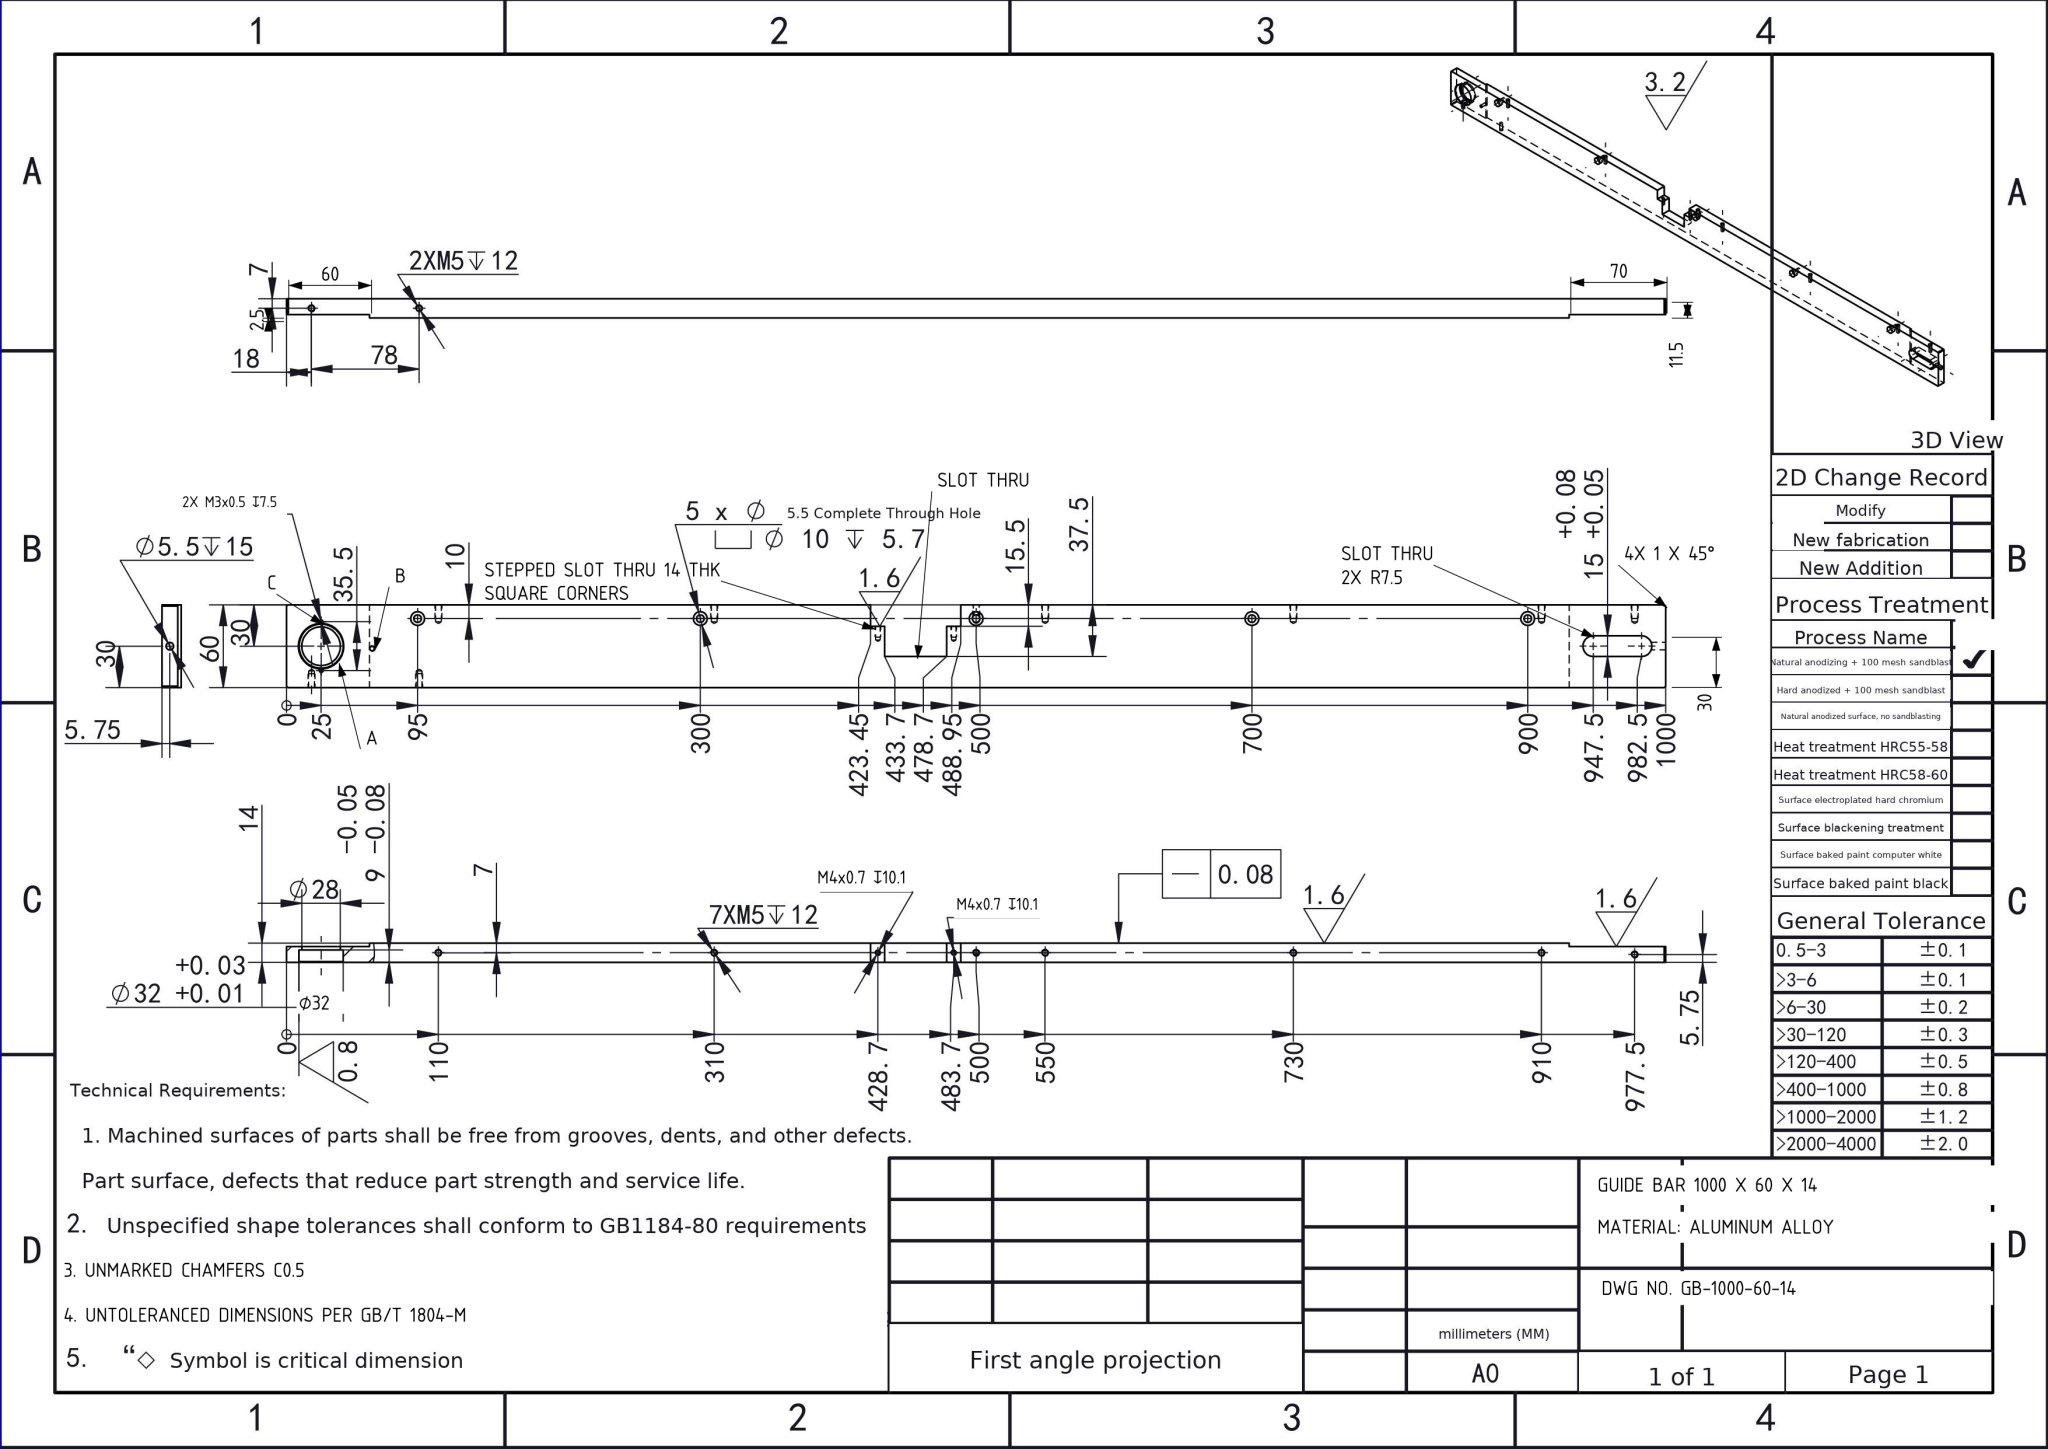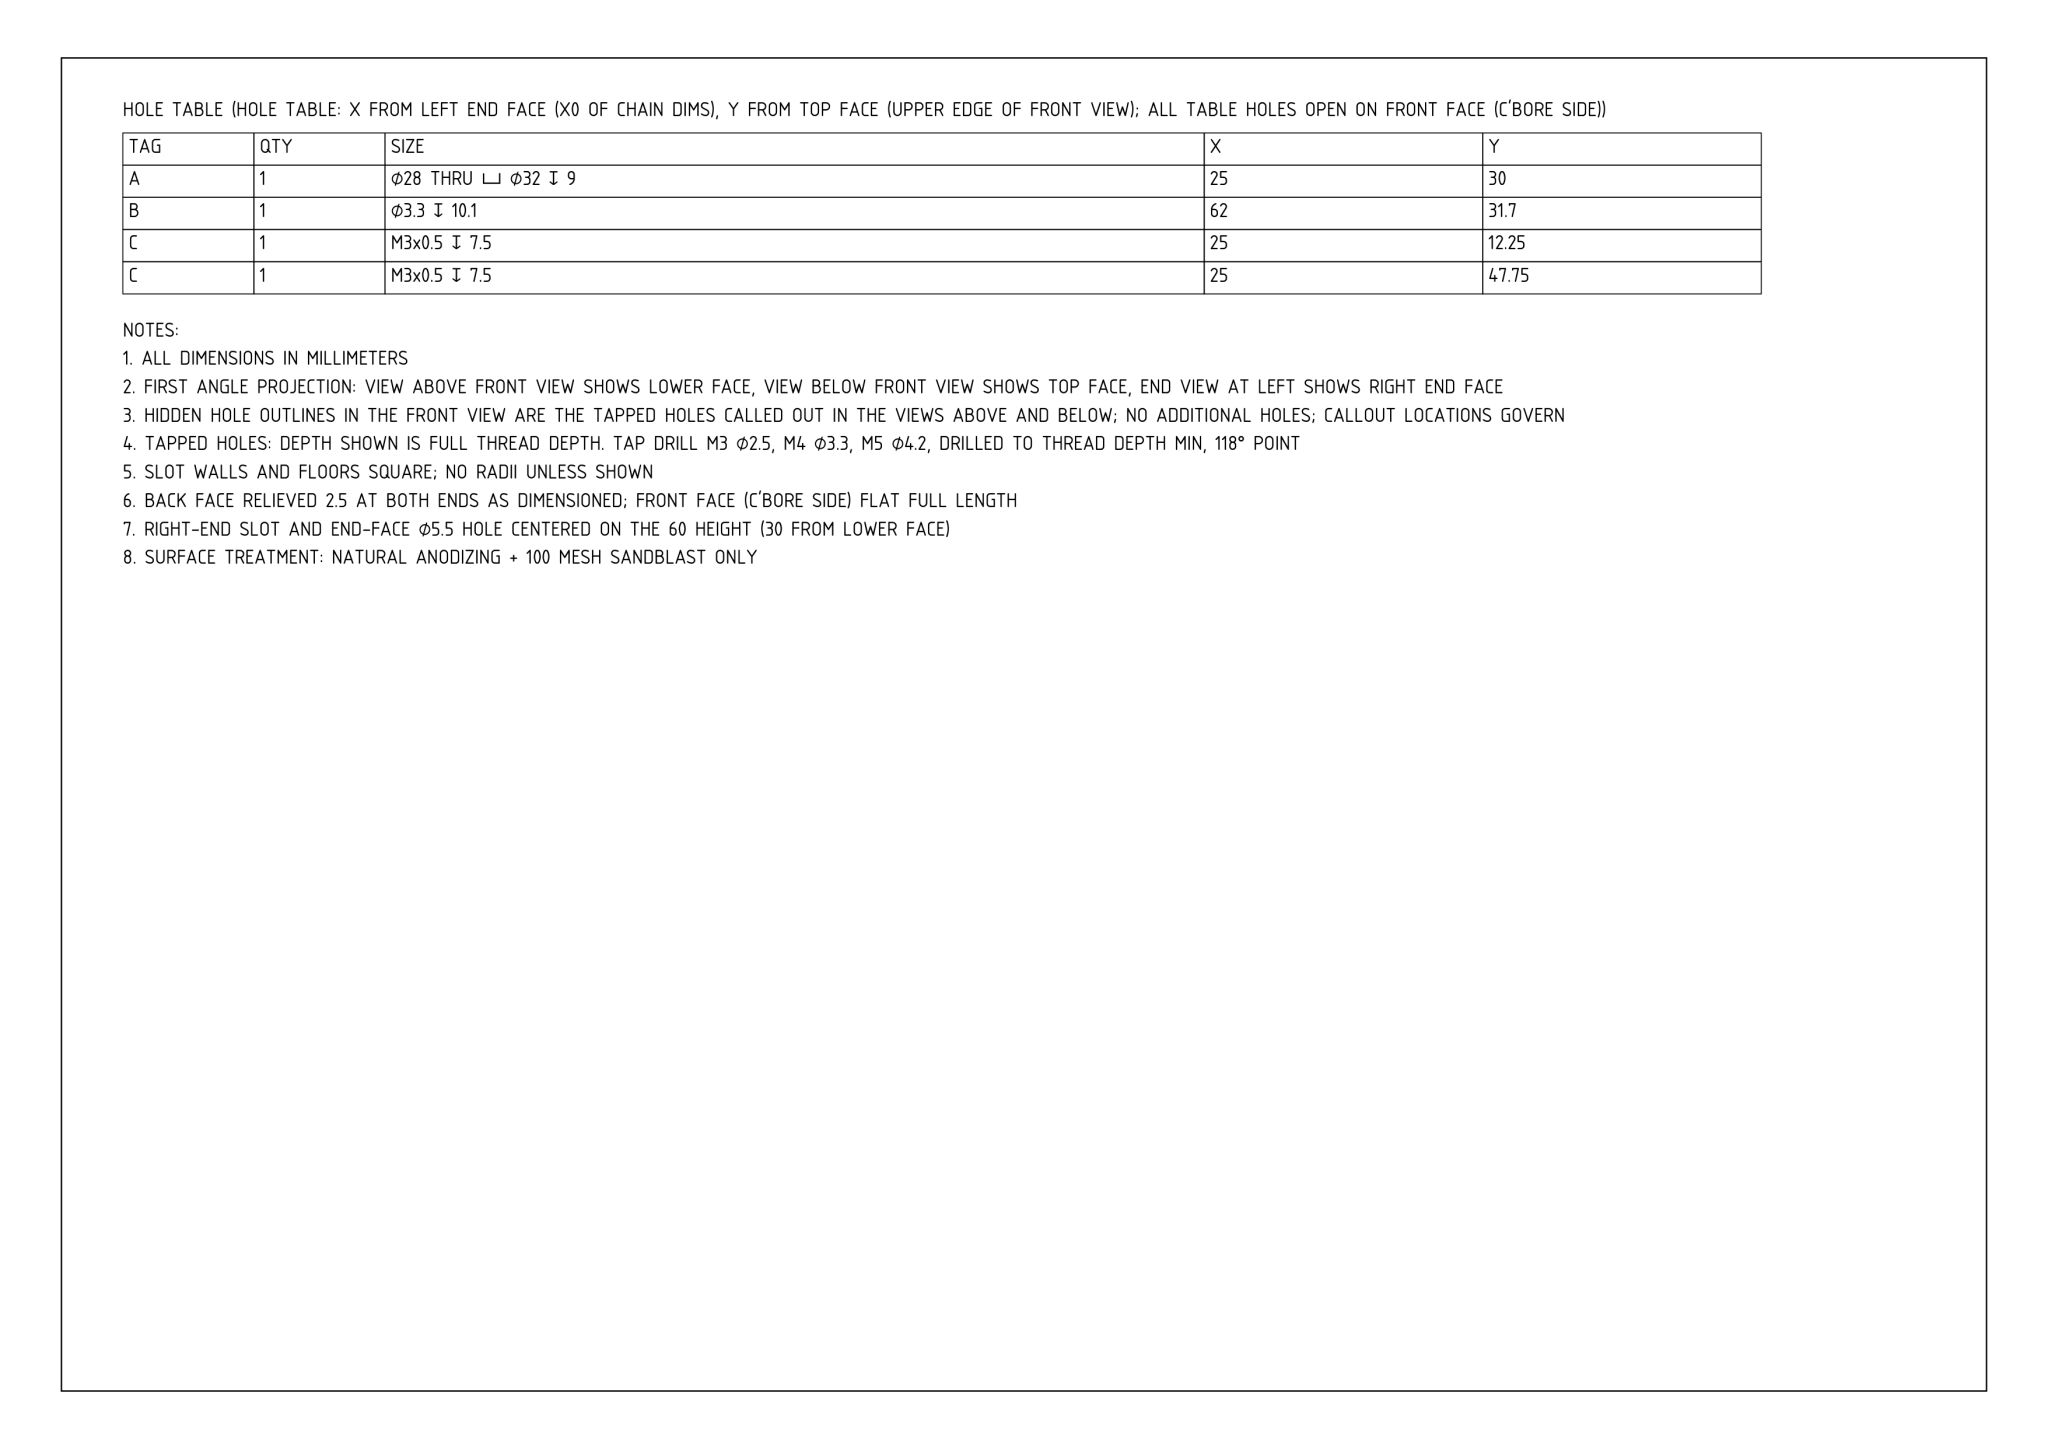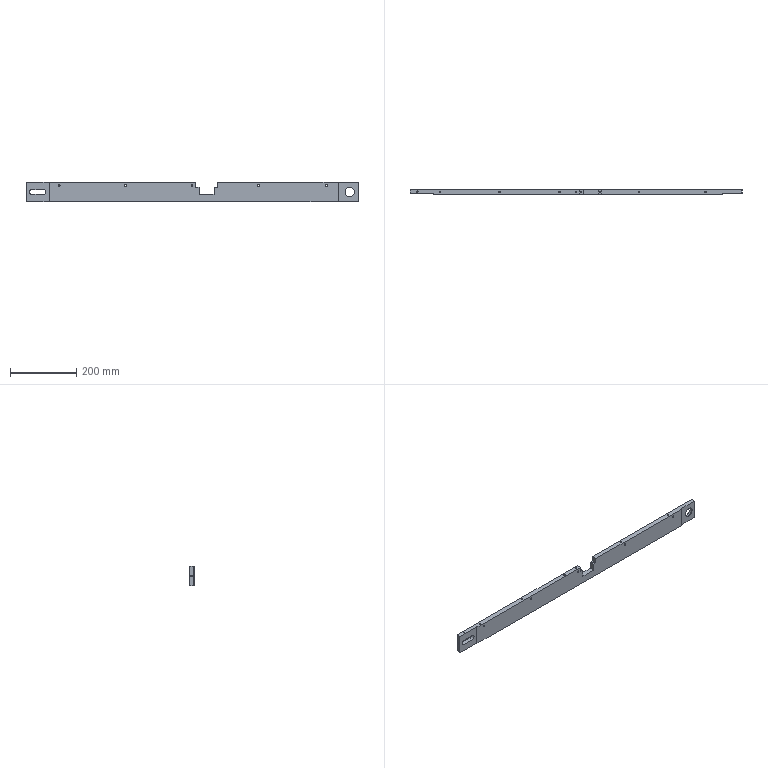Part | NX | mm | 1 solid | 119 faces | box 1000 x 14 x 60 mm | volume 770221 mm3 | cylinder 59 | cone 30 | plane 30 | commonest cylinder face diameters 4.2 x21 5.5 x12 10 x10 3.3 x6 2.5 x4 32 x2 28 x2 15 x2